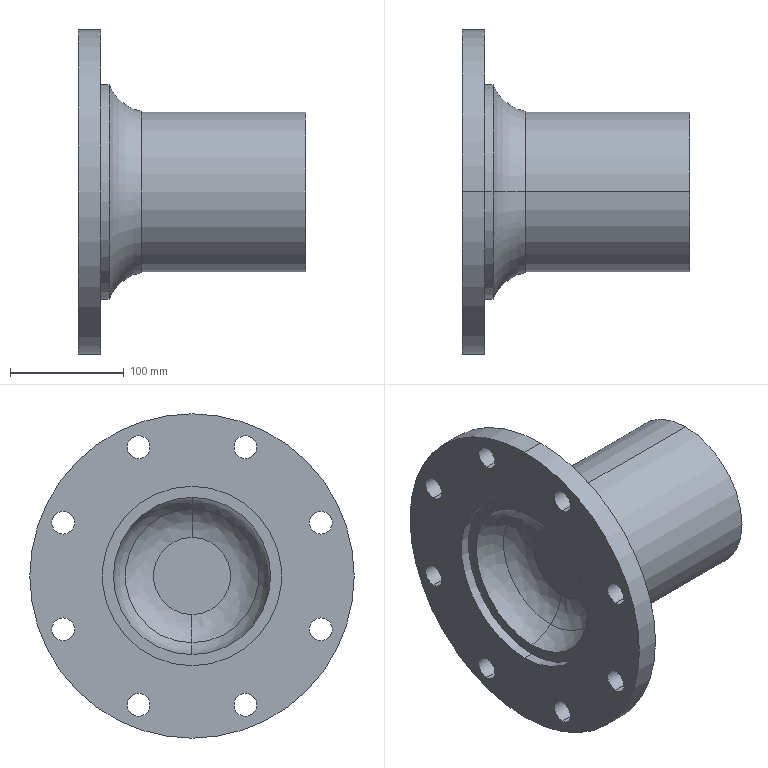Component | NX | BRIDA2_587_PREDETERMINADO_COMO_MECANIZADA_2 | 1 solid | 41 faces | volume 2943550 mm3 | cylinder 26 | spline 6 | plane 5 | torus 2 | cone 2 | commonest cylinder face diameters 20.1 x16 140 x2 80 x2 157.541 x2 285 x2 188.837 x2